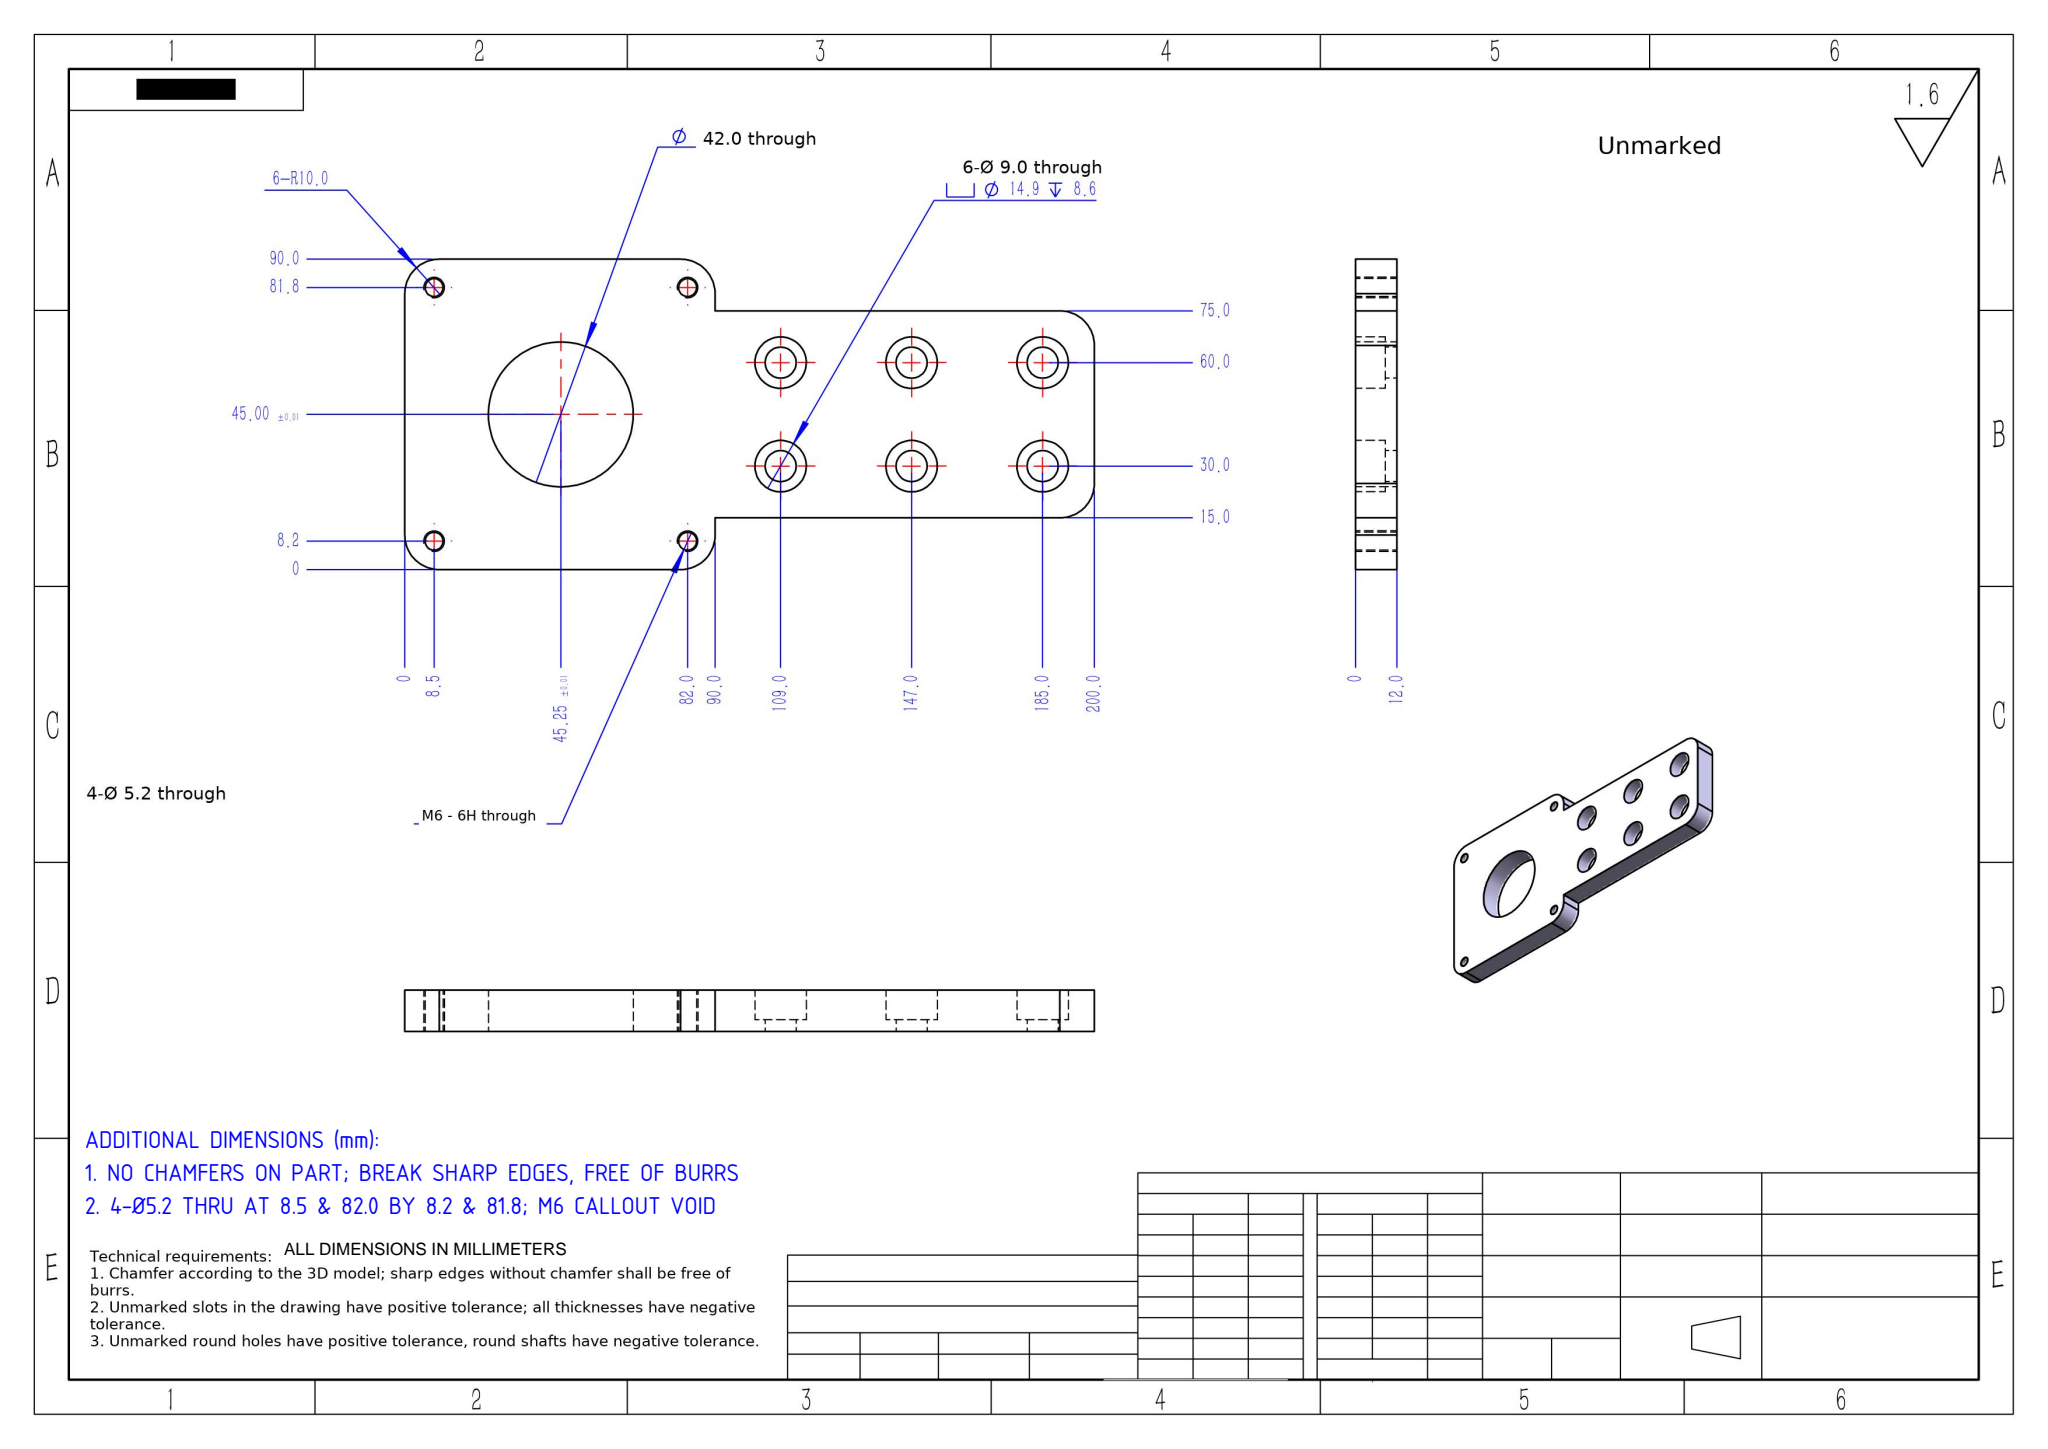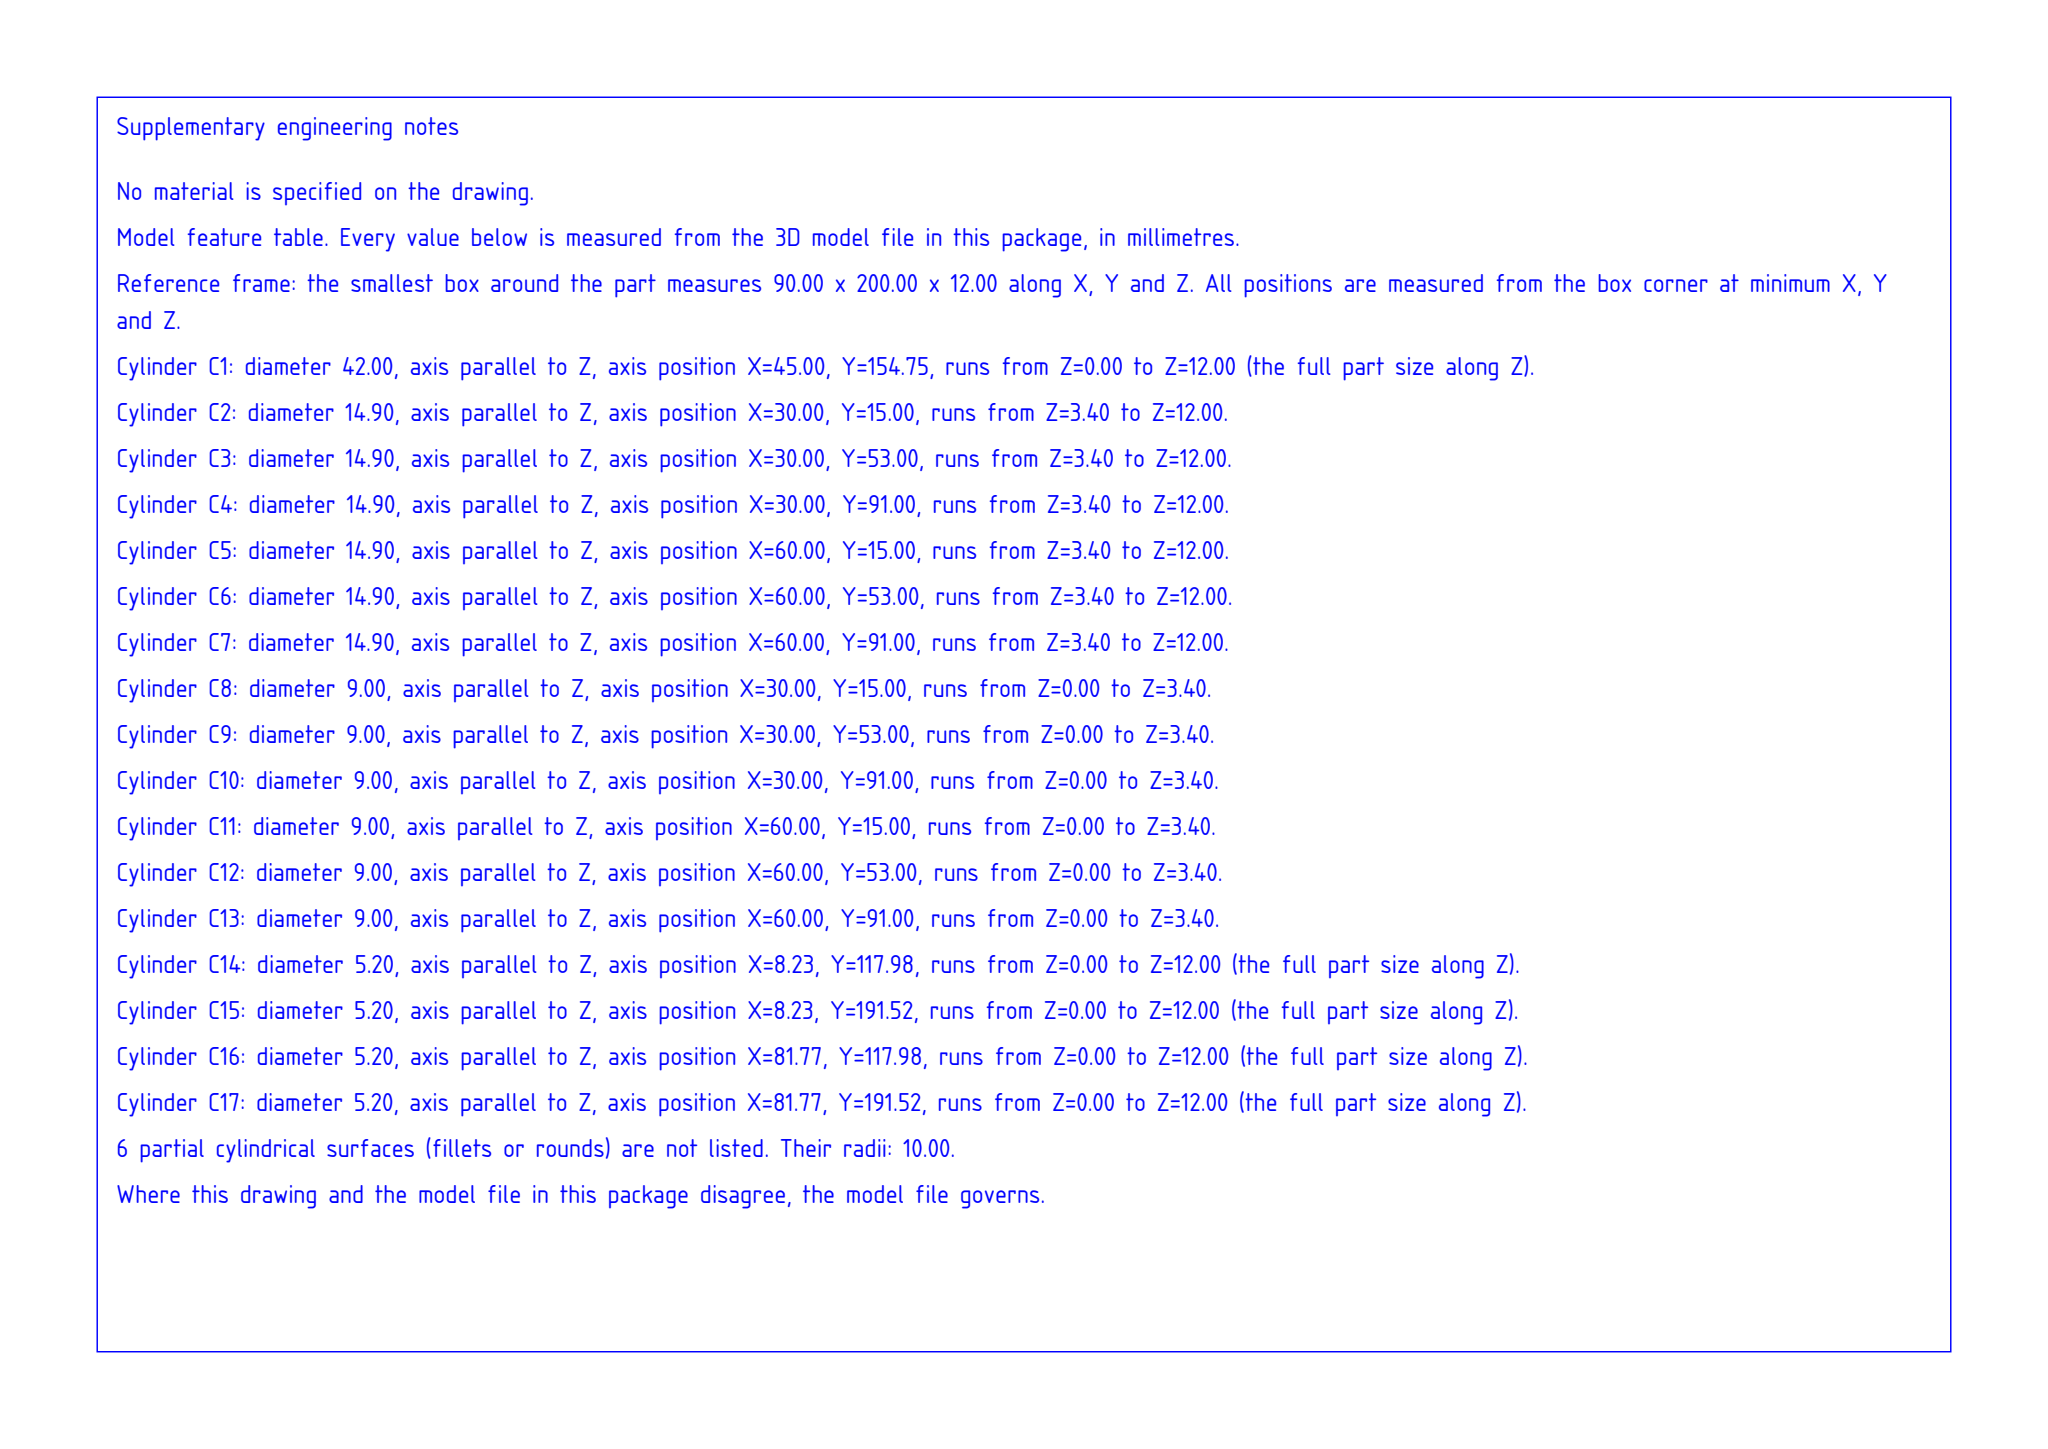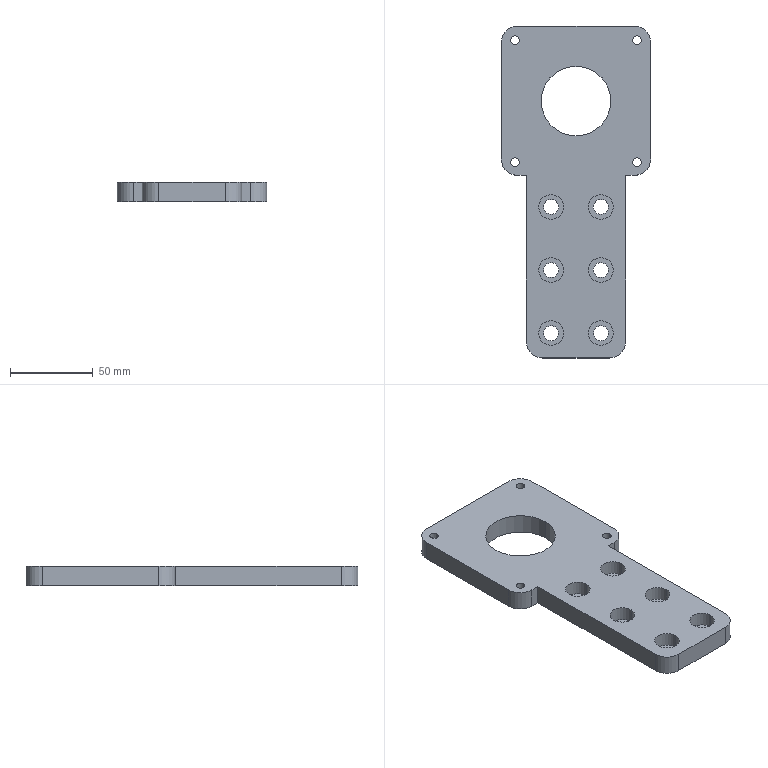Part | SolidWorks | mm | 1 solid | 56 faces | box 90 x 200 x 12 mm | volume 146915 mm3 | cylinder 40 | plane 16 | commonest cylinder face diameters 14.9 x12 9 x12 5.2 x8 20 x6 42 x2
build123d program:
from build123d import *

# Parameters (mm, degrees)
SKETCH1_W                                       = 90
SKETCH1_H                                       = 200
BOSS_EXTRUDE1_DEPTH                             = 6
FILLET1_R                                       = 10
SKETCH2_W                                       = 15
SKETCH2_H                                       = 110
CUT_EXTRUDE1_DEPTH                              = 111.313
FILLET2_R                                       = 10
FILLET3_R                                       = 10
SIZE_MM_DOWEL_HOLE1_D                           = 42
M8_HEX_SOCKET_HEAD_CAP_SCREW_CBORE1_D           = 9
M8_HEX_SOCKET_HEAD_CAP_SCREW_CBORE1_CBORE_D     = 14.9
M8_HEX_SOCKET_HEAD_CAP_SCREW_CBORE1_CBORE_DEPTH = 8.6
M6_TAPPED_HOLE1_D                               = 5.2


with BuildPart() as part:
    # Sketch1 → Boss-Extrude1 (new, symmetric)
    with BuildSketch(Plane.XY):
        Rectangle(SKETCH1_W, SKETCH1_H)
    extrude(amount=BOSS_EXTRUDE1_DEPTH, both=True)

    # Fillet1
    fillet1_edges = [part.edges().sort_by_distance(p)[0] for p in [
        (-45, 100, 0),
        (45, 100, 0),
    ]]
    fillet(fillet1_edges, radius=FILLET1_R)

    # Sketch2 → Cut-Extrude1 (cut, through all)
    with BuildSketch(Plane.XY.offset(6)):
        with Locations((-37.5, -45)):
            Rectangle(SKETCH2_W, SKETCH2_H)
    cut_extrude1 = extrude(amount=-CUT_EXTRUDE1_DEPTH, mode=Mode.SUBTRACT)

    # Mirror1: Cut-Extrude1 across plane
    add(cut_extrude1.mirror(Plane(origin=(0, 0, 0), x_dir=(0, 0, 1), z_dir=(1, 0, 0))), mode=Mode.SUBTRACT)

    # Fillet2
    fillet2_edges = [part.edges().sort_by_distance(p)[0] for p in [
        (-45, 10, 0),
        (45, 10, 0),
    ]]
    fillet(fillet2_edges, radius=FILLET2_R)

    # Fillet3
    fillet3_edges = [part.edges().sort_by_distance(p)[0] for p in [
        (-30, -100, 0),
        (30, -100, 0),
    ]]
    fillet(fillet3_edges, radius=FILLET3_R)

    # Size mm Dowel Hole1 (through all)
    with Locations(Plane.XY.offset(6)):
        with Locations((0, 54.75)):
            Hole(SIZE_MM_DOWEL_HOLE1_D / 2)

    # M8 Hex Socket Head Cap Screw CBORE1 (through all)
    with Locations(Plane.XY.offset(6)):
        with Locations((-15, -85), (-15, -47), (-15, -9)):
            m8_hex_socket_head_cap_screw_cbore1 = CounterBoreHole(M8_HEX_SOCKET_HEAD_CAP_SCREW_CBORE1_D / 2, M8_HEX_SOCKET_HEAD_CAP_SCREW_CBORE1_CBORE_D / 2, M8_HEX_SOCKET_HEAD_CAP_SCREW_CBORE1_CBORE_DEPTH)

    # Mirror2: M8 Hex Socket Head Cap Screw CBORE1 across plane
    add(m8_hex_socket_head_cap_screw_cbore1.mirror(Plane(origin=(0, 0, 0), x_dir=(0, 0, 1), z_dir=(1, 0, 0))), mode=Mode.SUBTRACT)

    # M6 Tapped Hole1 (through all)
    with Locations(Plane.XY.offset(6)):
        with Locations((36.77, 17.98), (36.77, 91.52), (-36.77, 91.52), (-36.77, 17.98)):
            Hole(M6_TAPPED_HOLE1_D / 2)


solid = part.part